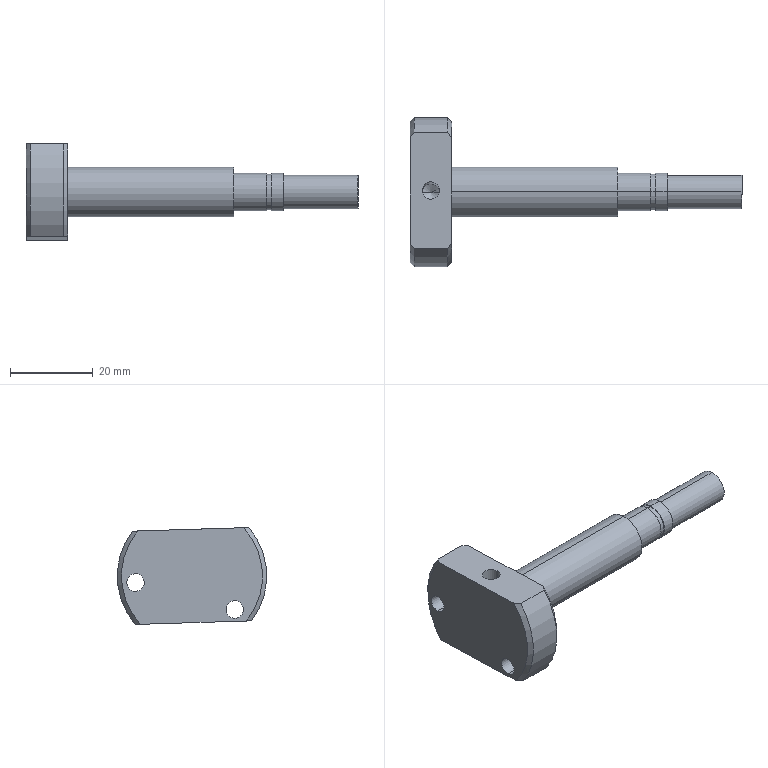Component | SolidWorks | CylinderConnectionPlate-1 | 1 solid | 39 faces | box 80 x 36 x 23.36 mm | volume 12759 mm3 | cylinder 22 | plane 9 | cone 8 | commonest cylinder face diameters 4.2 x8 9 x4 8.6 x2 2.291 x2 8 x2 12 x2 36 x2
build123d program:
from build123d import *

# Parameters (mm, degrees)
BOSS_EXTRUDE1_DEPTH     = 10
CHAMFER1_SIZE           = 1
M5_TAPPED_HOLE1_D       = 4.2
M5_TAPPED_HOLE1_DEPTH   = 15
M5_TAPPED_HOLE1_TIP     = 1.262
SKETCH11_R              = 6
BOSS_EXTRUDE2_DEPTH     = 40
SKETCH12_R              = 4.5
BOSS_EXTRUDE3_DEPTH     = 12
SKETCH13_R              = 4
BOSS_EXTRUDE4_DEPTH     = 18
CUT_EXTRUDE1_REACH      = 84.768
CUT_EXTRUDE1_END_RADIUS = 2.1
SKETCH14_R              = 1.146
M5_TAPPED_HOLE2_D       = 4.2
M5_TAPPED_HOLE2_DEPTH   = 12.4
M5_TAPPED_HOLE2_TIP     = 1.262
SKETCH17_W              = 1.15
SKETCH17_H              = 0.2
M5_TAPPED_HOLE3_D       = 4.2


with BuildPart() as part:
    # Sketch1 → Boss-Extrude1 (new body)
    with BuildSketch(Plane.XY):
        with BuildLine():
            Line((-11.25, -14.051), (-11.25, 14.051))
            ThreePointArc((-11.25, 14.051), (0, 18), (11.25, 14.051))
            Line((11.25, 14.051), (11.25, -14.051))
            ThreePointArc((11.25, -14.051), (0, -18), (-11.25, -14.051))
        make_face()
    extrude(amount=BOSS_EXTRUDE1_DEPTH)

    # Chamfer1
    chamfer1_edges = [part.edges().sort_by_distance(p)[0] for p in [
        (0, 18, 10),
        (0, -18, 10),
        (0, 18, 0),
        (0, -18, 0),
    ]]
    chamfer(chamfer1_edges, length=CHAMFER1_SIZE)

    # M5 Tapped Hole1
    with Locations(Plane.ZY.offset(11.25)):
        with Locations((5, 0)):
            Hole(M5_TAPPED_HOLE1_D / 2, depth=M5_TAPPED_HOLE1_DEPTH)
            with Locations((0, 0, -(M5_TAPPED_HOLE1_DEPTH + M5_TAPPED_HOLE1_TIP / 2))):  # 118° drill point
                Cone(0, M5_TAPPED_HOLE1_D / 2, M5_TAPPED_HOLE1_TIP, mode=Mode.SUBTRACT)

    # Sketch11 → Boss-Extrude2 (add)
    with BuildSketch(Plane.XY.offset(10)):
        Circle(SKETCH11_R)
    extrude(amount=BOSS_EXTRUDE2_DEPTH)

    # Sketch12 → Boss-Extrude3 (add)
    with BuildSketch(Plane.XY.offset(50)):
        Circle(SKETCH12_R)
    extrude(amount=BOSS_EXTRUDE3_DEPTH)

    # Sketch13 → Boss-Extrude4 (add)
    with BuildSketch(Plane.XY.offset(62)):
        Circle(SKETCH13_R)
    extrude(amount=BOSS_EXTRUDE4_DEPTH)

    # Cut-Extrude1: up to this cylinder (the profile starts outside it)
    cut_extrude1_end = Plane(origin=(0, 0, 5), z_dir=(-1, 0, 0)) * Cylinder(CUT_EXTRUDE1_END_RADIUS, 174.736, mode=Mode.PRIVATE)
    # Sketch14 → Cut-Extrude1 (cut, up to the surface)
    with BuildSketch(Plane.XY.offset(80), mode=Mode.PRIVATE) as cut_extrude1_sk1:
        Circle(SKETCH14_R)
    cut_extrude1_tool1 = extrude(cut_extrude1_sk1.sketch, amount=-CUT_EXTRUDE1_REACH, mode=Mode.PRIVATE) - cut_extrude1_end
    add(cut_extrude1_tool1.solids().sort_by_distance((0, 0, 80))[0], mode=Mode.SUBTRACT)

    # M5 Tapped Hole2
    with Locations(Plane.XY.offset(80)):
        with Locations((0, 0)):
            Hole(M5_TAPPED_HOLE2_D / 2, depth=M5_TAPPED_HOLE2_DEPTH)
            with Locations((0, 0, -(M5_TAPPED_HOLE2_DEPTH + M5_TAPPED_HOLE2_TIP / 2))):  # 118° drill point
                Cone(0, M5_TAPPED_HOLE2_D / 2, M5_TAPPED_HOLE2_TIP, mode=Mode.SUBTRACT)

    # Sketch17 → Cut-Revolve1 (revolve, cut)
    with BuildSketch(Plane(origin=(0, 0, 0), x_dir=(0, 0, -1), z_dir=(1, 0, 0)), mode=Mode.PRIVATE) as cut_revolve1_sk:
        with Locations((-58.575, 4.4)):
            Rectangle(SKETCH17_W, SKETCH17_H)
    revolve(cut_revolve1_sk.sketch.rotate(Axis((0, 0, 0), (0, 0, 1)), 90), axis=Axis((0, 0, 0), (0, 0, 1)), mode=Mode.SUBTRACT)

    # M5 Tapped Hole3 (through all)
    with Locations(Plane(origin=(0, 0, 0), x_dir=(-1, 0, 0), z_dir=(0, 0, -1))):
        with Locations((-1.144, 13.646), (-8.381, -10.032)):
            Hole(M5_TAPPED_HOLE3_D / 2)


solid = part.part

# Placed as in the assembly
solid = solid.moved(Location((-86.695, 50.945, -97.449), (-1.779, 90, 0)))